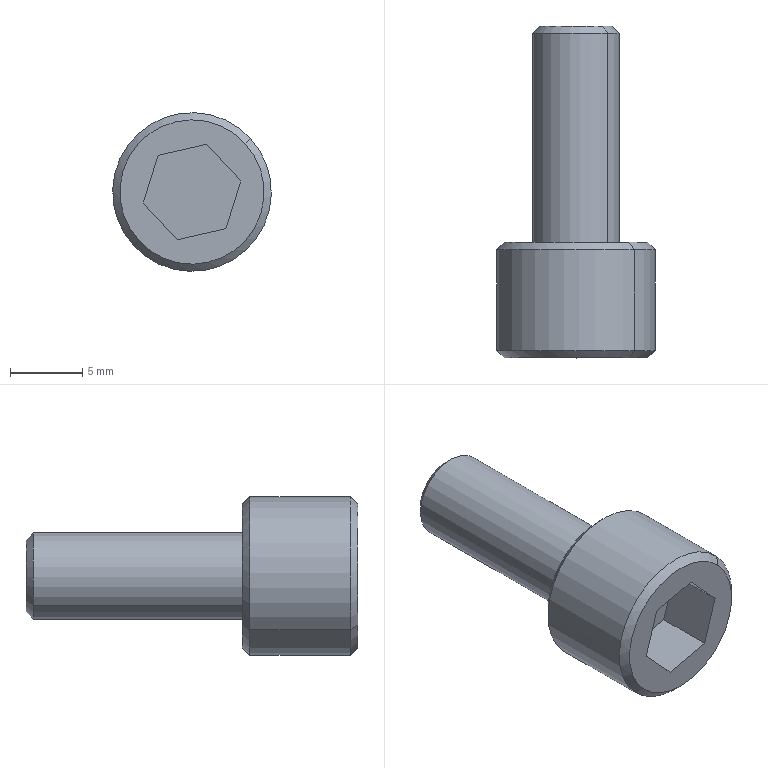Component | SolidWorks | 21-2 | 1 solid | 20 faces | box 11 x 23 x 11 mm | volume 1049 mm3 | plane 10 | cone 6 | cylinder 4 | commonest cylinder face diameters 6 x2 11 x2
STEP:
#1=CARTESIAN_POINT('',(-1.266,-2.358,0.6222));
#2=VERTEX_POINT('',#1);
#3=CARTESIAN_POINT('',(-1.121,-2.358,0.7558));
#4=VERTEX_POINT('',#3);
#5=CARTESIAN_POINT('',(-1.193,-2.358,0.689));
#6=DIRECTION('',(0.,1.,-0.));
#7=DIRECTION('',(-0.7345,0.,-0.6786));
#8=AXIS2_PLACEMENT_3D('',#5,#6,#7);
#9=CIRCLE('',#8,0.09843);
#10=EDGE_CURVE('',#2,#4,#9,.T.);
#11=ORIENTED_EDGE('',*,*,#10,.F.);
#12=CARTESIAN_POINT('',(-1.28,-2.377,0.6088));
#13=VERTEX_POINT('',#12);
#14=CARTESIAN_POINT('',(-1.266,-2.358,0.6222));
#15=DIRECTION('',(-0.5194,-0.7071,-0.4798));
#16=VECTOR('',#15,39.37);
#17=LINE('',#14,#16);
#18=EDGE_CURVE('',#2,#13,#17,.T.);
#19=ORIENTED_EDGE('',*,*,#18,.T.);
#20=CARTESIAN_POINT('',(-1.107,-2.377,0.7691));
#21=VERTEX_POINT('',#20);
#22=CARTESIAN_POINT('',(-1.193,-2.377,0.689));
#23=DIRECTION('',(-0.,-1.,0.));
#24=DIRECTION('',(-0.7345,0.,-0.6786));
#25=AXIS2_PLACEMENT_3D('',#22,#23,#24);
#26=CIRCLE('',#25,0.1181);
#27=EDGE_CURVE('',#21,#13,#26,.T.);
#28=ORIENTED_EDGE('',*,*,#27,.F.);
#29=CARTESIAN_POINT('',(-1.121,-2.358,0.7558));
#30=DIRECTION('',(0.5194,-0.7071,0.4798));
#31=VECTOR('',#30,39.37);
#32=LINE('',#29,#31);
#33=EDGE_CURVE('',#4,#21,#32,.T.);
#34=ORIENTED_EDGE('',*,*,#33,.F.);
#35=EDGE_LOOP('',(#11,#19,#28,#34));
#36=FACE_OUTER_BOUND('',#35,.T.);
#37=CARTESIAN_POINT('',(-1.193,-2.358,0.689));
#38=DIRECTION('',(-0.,-1.,0.));
#39=DIRECTION('',(0.7345,0.,0.6786));
#40=AXIS2_PLACEMENT_3D('',#37,#38,#39);
#41=CONICAL_SURFACE('',#40,0.09843,0.7854);
#42=ADVANCED_FACE('',(#36),#41,.T.);
#43=CARTESIAN_POINT('',(-1.338,-2.948,0.5554));
#44=VERTEX_POINT('',#43);
#45=CARTESIAN_POINT('',(-1.049,-2.948,0.8226));
#46=VERTEX_POINT('',#45);
#47=CARTESIAN_POINT('',(-1.193,-2.948,0.689));
#48=DIRECTION('',(0.,1.,-0.));
#49=DIRECTION('',(-0.7345,0.,-0.6786));
#50=AXIS2_PLACEMENT_3D('',#47,#48,#49);
#51=CIRCLE('',#50,0.1969);
#52=EDGE_CURVE('',#44,#46,#51,.T.);
#53=ORIENTED_EDGE('',*,*,#52,.F.);
#54=CARTESIAN_POINT('',(-1.352,-2.968,0.542));
#55=VERTEX_POINT('',#54);
#56=CARTESIAN_POINT('',(-1.338,-2.948,0.5554));
#57=DIRECTION('',(-0.5194,-0.7071,-0.4798));
#58=VECTOR('',#57,39.37);
#59=LINE('',#56,#58);
#60=EDGE_CURVE('',#44,#55,#59,.T.);
#61=ORIENTED_EDGE('',*,*,#60,.T.);
#62=CARTESIAN_POINT('',(-1.034,-2.968,0.8359));
#63=VERTEX_POINT('',#62);
#64=CARTESIAN_POINT('',(-1.193,-2.968,0.689));
#65=DIRECTION('',(-0.,-1.,0.));
#66=DIRECTION('',(-0.7345,0.,-0.6786));
#67=AXIS2_PLACEMENT_3D('',#64,#65,#66);
#68=CIRCLE('',#67,0.2165);
#69=EDGE_CURVE('',#63,#55,#68,.T.);
#70=ORIENTED_EDGE('',*,*,#69,.F.);
#71=CARTESIAN_POINT('',(-1.049,-2.948,0.8226));
#72=DIRECTION('',(0.5194,-0.7071,0.4798));
#73=VECTOR('',#72,39.37);
#74=LINE('',#71,#73);
#75=EDGE_CURVE('',#46,#63,#74,.T.);
#76=ORIENTED_EDGE('',*,*,#75,.F.);
#77=EDGE_LOOP('',(#53,#61,#70,#76));
#78=FACE_OUTER_BOUND('',#77,.T.);
#79=CARTESIAN_POINT('',(-1.193,-2.948,0.689));
#80=DIRECTION('',(-0.,-1.,0.));
#81=DIRECTION('',(0.7345,0.,0.6786));
#82=AXIS2_PLACEMENT_3D('',#79,#80,#81);
#83=CONICAL_SURFACE('',#82,0.1969,0.7854);
#84=ADVANCED_FACE('',(#78),#83,.T.);
#85=CARTESIAN_POINT('',(-1.049,-3.263,0.8226));
#86=VERTEX_POINT('',#85);
#87=CARTESIAN_POINT('',(-1.338,-3.263,0.5554));
#88=VERTEX_POINT('',#87);
#89=CARTESIAN_POINT('',(-1.193,-3.263,0.689));
#90=DIRECTION('',(-0.,-1.,0.));
#91=DIRECTION('',(-0.7345,0.,-0.6786));
#92=AXIS2_PLACEMENT_3D('',#89,#90,#91);
#93=CIRCLE('',#92,0.1969);
#94=EDGE_CURVE('',#86,#88,#93,.T.);
#95=ORIENTED_EDGE('',*,*,#94,.F.);
#96=CARTESIAN_POINT('',(-1.034,-3.243,0.8359));
#97=VERTEX_POINT('',#96);
#98=CARTESIAN_POINT('',(-1.034,-3.243,0.8359));
#99=DIRECTION('',(0.5194,0.7071,0.4798));
#100=VECTOR('',#99,39.37);
#101=LINE('',#98,#100);
#102=EDGE_CURVE('',#86,#97,#101,.T.);
#103=ORIENTED_EDGE('',*,*,#102,.T.);
#104=CARTESIAN_POINT('',(-1.352,-3.243,0.542));
#105=VERTEX_POINT('',#104);
#106=CARTESIAN_POINT('',(-1.193,-3.243,0.689));
#107=DIRECTION('',(0.,1.,-0.));
#108=DIRECTION('',(-0.7345,0.,-0.6786));
#109=AXIS2_PLACEMENT_3D('',#106,#107,#108);
#110=CIRCLE('',#109,0.2165);
#111=EDGE_CURVE('',#105,#97,#110,.T.);
#112=ORIENTED_EDGE('',*,*,#111,.F.);
#113=CARTESIAN_POINT('',(-1.352,-3.243,0.542));
#114=DIRECTION('',(-0.5194,0.7071,-0.4798));
#115=VECTOR('',#114,39.37);
#116=LINE('',#113,#115);
#117=EDGE_CURVE('',#88,#105,#116,.T.);
#118=ORIENTED_EDGE('',*,*,#117,.F.);
#119=EDGE_LOOP('',(#95,#103,#112,#118));
#120=FACE_OUTER_BOUND('',#119,.T.);
#121=CARTESIAN_POINT('',(-1.193,-3.243,0.689));
#122=DIRECTION('',(0.,1.,-0.));
#123=DIRECTION('',(-0.7345,0.,-0.6786));
#124=AXIS2_PLACEMENT_3D('',#121,#122,#123);
#125=CONICAL_SURFACE('',#124,0.2165,0.7854);
#126=ADVANCED_FACE('',(#120),#125,.T.);
#127=ORIENTED_EDGE('',*,*,#27,.T.);
#128=CARTESIAN_POINT('',(-1.28,-2.948,0.6088));
#129=VERTEX_POINT('',#128);
#130=CARTESIAN_POINT('',(-1.28,-2.358,0.6088));
#131=DIRECTION('',(-0.,-1.,0.));
#132=VECTOR('',#131,39.37);
#133=LINE('',#130,#132);
#134=EDGE_CURVE('',#13,#129,#133,.T.);
#135=ORIENTED_EDGE('',*,*,#134,.T.);
#136=CARTESIAN_POINT('',(-1.107,-2.948,0.7691));
#137=VERTEX_POINT('',#136);
#138=CARTESIAN_POINT('',(-1.193,-2.948,0.689));
#139=DIRECTION('',(0.,1.,-0.));
#140=DIRECTION('',(-0.7345,0.,-0.6786));
#141=AXIS2_PLACEMENT_3D('',#138,#139,#140);
#142=CIRCLE('',#141,0.1181);
#143=EDGE_CURVE('',#129,#137,#142,.T.);
#144=ORIENTED_EDGE('',*,*,#143,.T.);
#145=CARTESIAN_POINT('',(-1.107,-2.358,0.7691));
#146=DIRECTION('',(-0.,-1.,0.));
#147=VECTOR('',#146,39.37);
#148=LINE('',#145,#147);
#149=EDGE_CURVE('',#21,#137,#148,.T.);
#150=ORIENTED_EDGE('',*,*,#149,.F.);
#151=EDGE_LOOP('',(#127,#135,#144,#150));
#152=FACE_OUTER_BOUND('',#151,.T.);
#153=CARTESIAN_POINT('',(-1.193,-2.358,0.689));
#154=DIRECTION('',(-0.,-1.,0.));
#155=DIRECTION('',(0.7345,0.,0.6786));
#156=AXIS2_PLACEMENT_3D('',#153,#154,#155);
#157=CYLINDRICAL_SURFACE('',#156,0.1181);
#158=ADVANCED_FACE('',(#152),#157,.T.);
#159=ORIENTED_EDGE('',*,*,#69,.T.);
#160=CARTESIAN_POINT('',(-1.352,-2.948,0.542));
#161=DIRECTION('',(-0.,-1.,0.));
#162=VECTOR('',#161,39.37);
#163=LINE('',#160,#162);
#164=EDGE_CURVE('',#55,#105,#163,.T.);
#165=ORIENTED_EDGE('',*,*,#164,.T.);
#166=ORIENTED_EDGE('',*,*,#111,.T.);
#167=CARTESIAN_POINT('',(-1.034,-2.948,0.8359));
#168=DIRECTION('',(-0.,-1.,0.));
#169=VECTOR('',#168,39.37);
#170=LINE('',#167,#169);
#171=EDGE_CURVE('',#63,#97,#170,.T.);
#172=ORIENTED_EDGE('',*,*,#171,.F.);
#173=EDGE_LOOP('',(#159,#165,#166,#172));
#174=FACE_OUTER_BOUND('',#173,.T.);
#175=CARTESIAN_POINT('',(-1.193,-2.948,0.689));
#176=DIRECTION('',(-0.,-1.,0.));
#177=DIRECTION('',(0.7345,0.,0.6786));
#178=AXIS2_PLACEMENT_3D('',#175,#176,#177);
#179=CYLINDRICAL_SURFACE('',#178,0.2165);
#180=ADVANCED_FACE('',(#174),#179,.T.);
#181=ORIENTED_EDGE('',*,*,#164,.F.);
#182=CARTESIAN_POINT('',(-1.193,-2.968,0.689));
#183=DIRECTION('',(-0.,-1.,0.));
#184=DIRECTION('',(-0.7345,0.,-0.6786));
#185=AXIS2_PLACEMENT_3D('',#182,#183,#184);
#186=CIRCLE('',#185,0.2165);
#187=EDGE_CURVE('',#55,#63,#186,.T.);
#188=ORIENTED_EDGE('',*,*,#187,.T.);
#189=ORIENTED_EDGE('',*,*,#171,.T.);
#190=CARTESIAN_POINT('',(-1.193,-3.243,0.689));
#191=DIRECTION('',(0.,1.,-0.));
#192=DIRECTION('',(-0.7345,0.,-0.6786));
#193=AXIS2_PLACEMENT_3D('',#190,#191,#192);
#194=CIRCLE('',#193,0.2165);
#195=EDGE_CURVE('',#97,#105,#194,.T.);
#196=ORIENTED_EDGE('',*,*,#195,.T.);
#197=EDGE_LOOP('',(#181,#188,#189,#196));
#198=FACE_OUTER_BOUND('',#197,.T.);
#199=CARTESIAN_POINT('',(-1.193,-2.948,0.689));
#200=DIRECTION('',(-0.,-1.,0.));
#201=DIRECTION('',(0.7345,0.,0.6786));
#202=AXIS2_PLACEMENT_3D('',#199,#200,#201);
#203=CYLINDRICAL_SURFACE('',#202,0.2165);
#204=ADVANCED_FACE('',(#198),#203,.T.);
#205=CARTESIAN_POINT('',(-1.193,-2.948,0.689));
#206=DIRECTION('',(0.,1.,-0.));
#207=DIRECTION('',(-0.7345,0.,-0.6786));
#208=AXIS2_PLACEMENT_3D('',#205,#206,#207);
#209=CIRCLE('',#208,0.1969);
#210=EDGE_CURVE('',#46,#44,#209,.T.);
#211=ORIENTED_EDGE('',*,*,#210,.T.);
#212=ORIENTED_EDGE('',*,*,#52,.T.);
#213=EDGE_LOOP('',(#211,#212));
#214=FACE_OUTER_BOUND('',#213,.T.);
#215=CARTESIAN_POINT('',(-1.193,-2.948,0.689));
#216=DIRECTION('',(0.,1.,-0.));
#217=DIRECTION('',(-0.7345,0.,-0.6786));
#218=AXIS2_PLACEMENT_3D('',#215,#216,#217);
#219=CIRCLE('',#218,0.1181);
#220=EDGE_CURVE('',#137,#129,#219,.T.);
#221=ORIENTED_EDGE('',*,*,#220,.F.);
#222=ORIENTED_EDGE('',*,*,#143,.F.);
#223=EDGE_LOOP('',(#221,#222));
#224=FACE_BOUND('',#223,.T.);
#225=CARTESIAN_POINT('',(-1.193,-2.948,0.689));
#226=DIRECTION('',(0.,1.,-0.));
#227=DIRECTION('',(-0.7345,-0.,-0.6786));
#228=AXIS2_PLACEMENT_3D('',#225,#226,#227);
#229=PLANE('',#228);
#230=ADVANCED_FACE('',(#214,#224),#229,.T.);
#231=CARTESIAN_POINT('',(-1.06,-3.263,0.719));
#232=VERTEX_POINT('',#231);
#233=CARTESIAN_POINT('',(-1.153,-3.263,0.8192));
#234=VERTEX_POINT('',#233);
#235=CARTESIAN_POINT('',(-1.06,-3.263,0.719));
#236=DIRECTION('',(-0.6786,0.,0.7345));
#237=VECTOR('',#236,39.37);
#238=LINE('',#235,#237);
#239=EDGE_CURVE('',#232,#234,#238,.T.);
#240=ORIENTED_EDGE('',*,*,#239,.F.);
#241=CARTESIAN_POINT('',(-1.101,-3.263,0.5888));
#242=VERTEX_POINT('',#241);
#243=CARTESIAN_POINT('',(-1.101,-3.263,0.5888));
#244=DIRECTION('',(0.2968,0.,0.9549));
#245=VECTOR('',#244,39.37);
#246=LINE('',#243,#245);
#247=EDGE_CURVE('',#242,#232,#246,.T.);
#248=ORIENTED_EDGE('',*,*,#247,.F.);
#249=CARTESIAN_POINT('',(-1.234,-3.263,0.5587));
#250=VERTEX_POINT('',#249);
#251=CARTESIAN_POINT('',(-1.234,-3.263,0.5587));
#252=DIRECTION('',(0.9754,0.,0.2204));
#253=VECTOR('',#252,39.37);
#254=LINE('',#251,#253);
#255=EDGE_CURVE('',#250,#242,#254,.T.);
#256=ORIENTED_EDGE('',*,*,#255,.F.);
#257=CARTESIAN_POINT('',(-1.326,-3.263,0.6589));
#258=VERTEX_POINT('',#257);
#259=CARTESIAN_POINT('',(-1.326,-3.263,0.6589));
#260=DIRECTION('',(0.6786,-0.,-0.7345));
#261=VECTOR('',#260,39.37);
#262=LINE('',#259,#261);
#263=EDGE_CURVE('',#258,#250,#262,.T.);
#264=ORIENTED_EDGE('',*,*,#263,.F.);
#265=CARTESIAN_POINT('',(-1.286,-3.263,0.7892));
#266=VERTEX_POINT('',#265);
#267=CARTESIAN_POINT('',(-1.286,-3.263,0.7892));
#268=DIRECTION('',(-0.2968,-0.,-0.9549));
#269=VECTOR('',#268,39.37);
#270=LINE('',#267,#269);
#271=EDGE_CURVE('',#266,#258,#270,.T.);
#272=ORIENTED_EDGE('',*,*,#271,.F.);
#273=CARTESIAN_POINT('',(-1.153,-3.263,0.8192));
#274=DIRECTION('',(-0.9754,-0.,-0.2204));
#275=VECTOR('',#274,39.37);
#276=LINE('',#273,#275);
#277=EDGE_CURVE('',#234,#266,#276,.T.);
#278=ORIENTED_EDGE('',*,*,#277,.F.);
#279=EDGE_LOOP('',(#240,#248,#256,#264,#272,#278));
#280=FACE_BOUND('',#279,.T.);
#281=CARTESIAN_POINT('',(-1.193,-3.263,0.689));
#282=DIRECTION('',(-0.,-1.,0.));
#283=DIRECTION('',(-0.7345,0.,-0.6786));
#284=AXIS2_PLACEMENT_3D('',#281,#282,#283);
#285=CIRCLE('',#284,0.1969);
#286=EDGE_CURVE('',#88,#86,#285,.T.);
#287=ORIENTED_EDGE('',*,*,#286,.T.);
#288=ORIENTED_EDGE('',*,*,#94,.T.);
#289=EDGE_LOOP('',(#287,#288));
#290=FACE_OUTER_BOUND('',#289,.T.);
#291=CARTESIAN_POINT('',(-1.193,-3.263,0.689));
#292=DIRECTION('',(0.,1.,-0.));
#293=DIRECTION('',(-0.7345,-0.,-0.6786));
#294=AXIS2_PLACEMENT_3D('',#291,#292,#293);
#295=PLANE('',#294);
#296=ADVANCED_FACE('',(#280,#290),#295,.F.);
#297=ORIENTED_EDGE('',*,*,#134,.F.);
#298=CARTESIAN_POINT('',(-1.193,-2.377,0.689));
#299=DIRECTION('',(-0.,-1.,0.));
#300=DIRECTION('',(-0.7345,0.,-0.6786));
#301=AXIS2_PLACEMENT_3D('',#298,#299,#300);
#302=CIRCLE('',#301,0.1181);
#303=EDGE_CURVE('',#13,#21,#302,.T.);
#304=ORIENTED_EDGE('',*,*,#303,.T.);
#305=ORIENTED_EDGE('',*,*,#149,.T.);
#306=ORIENTED_EDGE('',*,*,#220,.T.);
#307=EDGE_LOOP('',(#297,#304,#305,#306));
#308=FACE_OUTER_BOUND('',#307,.T.);
#309=CARTESIAN_POINT('',(-1.193,-2.358,0.689));
#310=DIRECTION('',(-0.,-1.,0.));
#311=DIRECTION('',(0.7345,0.,0.6786));
#312=AXIS2_PLACEMENT_3D('',#309,#310,#311);
#313=CYLINDRICAL_SURFACE('',#312,0.1181);
#314=ADVANCED_FACE('',(#308),#313,.T.);
#315=CARTESIAN_POINT('',(-1.193,-2.358,0.689));
#316=DIRECTION('',(0.,1.,-0.));
#317=DIRECTION('',(-0.7345,0.,-0.6786));
#318=AXIS2_PLACEMENT_3D('',#315,#316,#317);
#319=CIRCLE('',#318,0.09843);
#320=EDGE_CURVE('',#4,#2,#319,.T.);
#321=ORIENTED_EDGE('',*,*,#320,.T.);
#322=ORIENTED_EDGE('',*,*,#10,.T.);
#323=EDGE_LOOP('',(#321,#322));
#324=FACE_OUTER_BOUND('',#323,.T.);
#325=CARTESIAN_POINT('',(-1.193,-2.358,0.689));
#326=DIRECTION('',(0.,1.,-0.));
#327=DIRECTION('',(-0.7345,-0.,-0.6786));
#328=AXIS2_PLACEMENT_3D('',#325,#326,#327);
#329=PLANE('',#328);
#330=ADVANCED_FACE('',(#324),#329,.T.);
#331=ORIENTED_EDGE('',*,*,#102,.F.);
#332=ORIENTED_EDGE('',*,*,#286,.F.);
#333=ORIENTED_EDGE('',*,*,#117,.T.);
#334=ORIENTED_EDGE('',*,*,#195,.F.);
#335=EDGE_LOOP('',(#331,#332,#333,#334));
#336=FACE_OUTER_BOUND('',#335,.T.);
#337=CARTESIAN_POINT('',(-1.193,-3.243,0.689));
#338=DIRECTION('',(0.,1.,-0.));
#339=DIRECTION('',(-0.7345,0.,-0.6786));
#340=AXIS2_PLACEMENT_3D('',#337,#338,#339);
#341=CONICAL_SURFACE('',#340,0.2165,0.7854);
#342=ADVANCED_FACE('',(#336),#341,.T.);
#343=ORIENTED_EDGE('',*,*,#60,.F.);
#344=ORIENTED_EDGE('',*,*,#210,.F.);
#345=ORIENTED_EDGE('',*,*,#75,.T.);
#346=ORIENTED_EDGE('',*,*,#187,.F.);
#347=EDGE_LOOP('',(#343,#344,#345,#346));
#348=FACE_OUTER_BOUND('',#347,.T.);
#349=CARTESIAN_POINT('',(-1.193,-2.948,0.689));
#350=DIRECTION('',(-0.,-1.,0.));
#351=DIRECTION('',(0.7345,0.,0.6786));
#352=AXIS2_PLACEMENT_3D('',#349,#350,#351);
#353=CONICAL_SURFACE('',#352,0.1969,0.7854);
#354=ADVANCED_FACE('',(#348),#353,.T.);
#355=ORIENTED_EDGE('',*,*,#18,.F.);
#356=ORIENTED_EDGE('',*,*,#320,.F.);
#357=ORIENTED_EDGE('',*,*,#33,.T.);
#358=ORIENTED_EDGE('',*,*,#303,.F.);
#359=EDGE_LOOP('',(#355,#356,#357,#358));
#360=FACE_OUTER_BOUND('',#359,.T.);
#361=CARTESIAN_POINT('',(-1.193,-2.358,0.689));
#362=DIRECTION('',(-0.,-1.,0.));
#363=DIRECTION('',(0.7345,0.,0.6786));
#364=AXIS2_PLACEMENT_3D('',#361,#362,#363);
#365=CONICAL_SURFACE('',#364,0.09843,0.7854);
#366=ADVANCED_FACE('',(#360),#365,.T.);
#367=ORIENTED_EDGE('',*,*,#247,.T.);
#368=CARTESIAN_POINT('',(-1.06,-3.106,0.719));
#369=VERTEX_POINT('',#368);
#370=CARTESIAN_POINT('',(-1.06,-3.106,0.719));
#371=DIRECTION('',(-0.,-1.,0.));
#372=VECTOR('',#371,39.37);
#373=LINE('',#370,#372);
#374=EDGE_CURVE('',#369,#232,#373,.T.);
#375=ORIENTED_EDGE('',*,*,#374,.F.);
#376=CARTESIAN_POINT('',(-1.101,-3.106,0.5888));
#377=VERTEX_POINT('',#376);
#378=CARTESIAN_POINT('',(-1.101,-3.106,0.5888));
#379=DIRECTION('',(0.2968,0.,0.9549));
#380=VECTOR('',#379,39.37);
#381=LINE('',#378,#380);
#382=EDGE_CURVE('',#377,#369,#381,.T.);
#383=ORIENTED_EDGE('',*,*,#382,.F.);
#384=CARTESIAN_POINT('',(-1.101,-3.106,0.5888));
#385=DIRECTION('',(-0.,-1.,0.));
#386=VECTOR('',#385,39.37);
#387=LINE('',#384,#386);
#388=EDGE_CURVE('',#377,#242,#387,.T.);
#389=ORIENTED_EDGE('',*,*,#388,.T.);
#390=EDGE_LOOP('',(#367,#375,#383,#389));
#391=FACE_OUTER_BOUND('',#390,.T.);
#392=CARTESIAN_POINT('',(-1.101,-3.106,0.5888));
#393=DIRECTION('',(0.9549,-0.,-0.2968));
#394=DIRECTION('',(-0.2968,-0.,-0.9549));
#395=AXIS2_PLACEMENT_3D('',#392,#393,#394);
#396=PLANE('',#395);
#397=ADVANCED_FACE('',(#391),#396,.F.);
#398=ORIENTED_EDGE('',*,*,#255,.T.);
#399=ORIENTED_EDGE('',*,*,#388,.F.);
#400=CARTESIAN_POINT('',(-1.234,-3.106,0.5587));
#401=VERTEX_POINT('',#400);
#402=CARTESIAN_POINT('',(-1.234,-3.106,0.5587));
#403=DIRECTION('',(0.9754,0.,0.2204));
#404=VECTOR('',#403,39.37);
#405=LINE('',#402,#404);
#406=EDGE_CURVE('',#401,#377,#405,.T.);
#407=ORIENTED_EDGE('',*,*,#406,.F.);
#408=CARTESIAN_POINT('',(-1.234,-3.106,0.5587));
#409=DIRECTION('',(-0.,-1.,0.));
#410=VECTOR('',#409,39.37);
#411=LINE('',#408,#410);
#412=EDGE_CURVE('',#401,#250,#411,.T.);
#413=ORIENTED_EDGE('',*,*,#412,.T.);
#414=EDGE_LOOP('',(#398,#399,#407,#413));
#415=FACE_OUTER_BOUND('',#414,.T.);
#416=CARTESIAN_POINT('',(-1.234,-3.106,0.5587));
#417=DIRECTION('',(0.2204,-0.,-0.9754));
#418=DIRECTION('',(-0.9754,-0.,-0.2204));
#419=AXIS2_PLACEMENT_3D('',#416,#417,#418);
#420=PLANE('',#419);
#421=ADVANCED_FACE('',(#415),#420,.F.);
#422=ORIENTED_EDGE('',*,*,#263,.T.);
#423=ORIENTED_EDGE('',*,*,#412,.F.);
#424=CARTESIAN_POINT('',(-1.326,-3.106,0.6589));
#425=VERTEX_POINT('',#424);
#426=CARTESIAN_POINT('',(-1.326,-3.106,0.6589));
#427=DIRECTION('',(0.6786,-0.,-0.7345));
#428=VECTOR('',#427,39.37);
#429=LINE('',#426,#428);
#430=EDGE_CURVE('',#425,#401,#429,.T.);
#431=ORIENTED_EDGE('',*,*,#430,.F.);
#432=CARTESIAN_POINT('',(-1.326,-3.106,0.6589));
#433=DIRECTION('',(-0.,-1.,0.));
#434=VECTOR('',#433,39.37);
#435=LINE('',#432,#434);
#436=EDGE_CURVE('',#425,#258,#435,.T.);
#437=ORIENTED_EDGE('',*,*,#436,.T.);
#438=EDGE_LOOP('',(#422,#423,#431,#437));
#439=FACE_OUTER_BOUND('',#438,.T.);
#440=CARTESIAN_POINT('',(-1.326,-3.106,0.6589));
#441=DIRECTION('',(-0.7345,-0.,-0.6786));
#442=DIRECTION('',(-0.6786,0.,0.7345));
#443=AXIS2_PLACEMENT_3D('',#440,#441,#442);
#444=PLANE('',#443);
#445=ADVANCED_FACE('',(#439),#444,.F.);
#446=ORIENTED_EDGE('',*,*,#271,.T.);
#447=ORIENTED_EDGE('',*,*,#436,.F.);
#448=CARTESIAN_POINT('',(-1.286,-3.106,0.7892));
#449=VERTEX_POINT('',#448);
#450=CARTESIAN_POINT('',(-1.286,-3.106,0.7892));
#451=DIRECTION('',(-0.2968,-0.,-0.9549));
#452=VECTOR('',#451,39.37);
#453=LINE('',#450,#452);
#454=EDGE_CURVE('',#449,#425,#453,.T.);
#455=ORIENTED_EDGE('',*,*,#454,.F.);
#456=CARTESIAN_POINT('',(-1.286,-3.106,0.7892));
#457=DIRECTION('',(-0.,-1.,0.));
#458=VECTOR('',#457,39.37);
#459=LINE('',#456,#458);
#460=EDGE_CURVE('',#449,#266,#459,.T.);
#461=ORIENTED_EDGE('',*,*,#460,.T.);
#462=EDGE_LOOP('',(#446,#447,#455,#461));
#463=FACE_OUTER_BOUND('',#462,.T.);
#464=CARTESIAN_POINT('',(-1.286,-3.106,0.7892));
#465=DIRECTION('',(-0.9549,0.,0.2968));
#466=DIRECTION('',(0.2968,0.,0.9549));
#467=AXIS2_PLACEMENT_3D('',#464,#465,#466);
#468=PLANE('',#467);
#469=ADVANCED_FACE('',(#463),#468,.F.);
#470=ORIENTED_EDGE('',*,*,#277,.T.);
#471=ORIENTED_EDGE('',*,*,#460,.F.);
#472=CARTESIAN_POINT('',(-1.153,-3.106,0.8192));
#473=VERTEX_POINT('',#472);
#474=CARTESIAN_POINT('',(-1.153,-3.106,0.8192));
#475=DIRECTION('',(-0.9754,-0.,-0.2204));
#476=VECTOR('',#475,39.37);
#477=LINE('',#474,#476);
#478=EDGE_CURVE('',#473,#449,#477,.T.);
#479=ORIENTED_EDGE('',*,*,#478,.F.);
#480=CARTESIAN_POINT('',(-1.153,-3.106,0.8192));
#481=DIRECTION('',(-0.,-1.,0.));
#482=VECTOR('',#481,39.37);
#483=LINE('',#480,#482);
#484=EDGE_CURVE('',#473,#234,#483,.T.);
#485=ORIENTED_EDGE('',*,*,#484,.T.);
#486=EDGE_LOOP('',(#470,#471,#479,#485));
#487=FACE_OUTER_BOUND('',#486,.T.);
#488=CARTESIAN_POINT('',(-1.153,-3.106,0.8192));
#489=DIRECTION('',(-0.2204,0.,0.9754));
#490=DIRECTION('',(0.9754,0.,0.2204));
#491=AXIS2_PLACEMENT_3D('',#488,#489,#490);
#492=PLANE('',#491);
#493=ADVANCED_FACE('',(#487),#492,.F.);
#494=ORIENTED_EDGE('',*,*,#239,.T.);
#495=ORIENTED_EDGE('',*,*,#484,.F.);
#496=CARTESIAN_POINT('',(-1.06,-3.106,0.719));
#497=DIRECTION('',(-0.6786,0.,0.7345));
#498=VECTOR('',#497,39.37);
#499=LINE('',#496,#498);
#500=EDGE_CURVE('',#369,#473,#499,.T.);
#501=ORIENTED_EDGE('',*,*,#500,.F.);
#502=ORIENTED_EDGE('',*,*,#374,.T.);
#503=EDGE_LOOP('',(#494,#495,#501,#502));
#504=FACE_OUTER_BOUND('',#503,.T.);
#505=CARTESIAN_POINT('',(-1.06,-3.106,0.719));
#506=DIRECTION('',(0.7345,0.,0.6786));
#507=DIRECTION('',(0.6786,-0.,-0.7345));
#508=AXIS2_PLACEMENT_3D('',#505,#506,#507);
#509=PLANE('',#508);
#510=ADVANCED_FACE('',(#504),#509,.F.);
#511=ORIENTED_EDGE('',*,*,#382,.T.);
#512=ORIENTED_EDGE('',*,*,#500,.T.);
#513=ORIENTED_EDGE('',*,*,#478,.T.);
#514=ORIENTED_EDGE('',*,*,#454,.T.);
#515=ORIENTED_EDGE('',*,*,#430,.T.);
#516=ORIENTED_EDGE('',*,*,#406,.T.);
#517=EDGE_LOOP('',(#511,#512,#513,#514,#515,#516));
#518=FACE_OUTER_BOUND('',#517,.T.);
#519=CARTESIAN_POINT('',(-1.193,-3.106,0.689));
#520=DIRECTION('',(-0.,-1.,0.));
#521=DIRECTION('',(0.7345,0.,0.6786));
#522=AXIS2_PLACEMENT_3D('',#519,#520,#521);
#523=PLANE('',#522);
#524=ADVANCED_FACE('',(#518),#523,.T.);
#525=CLOSED_SHELL('',(#42,#84,#126,#158,#180,#204,#230,#296,#314,#330,#342,#354,#366,#397,#421,#445,#469,#493,#510,#524));
#526=MANIFOLD_SOLID_BREP('',#525);
#527=CARTESIAN_POINT('',(0.,0.,0.));
#528=DIRECTION('',(0.,0.,1.));
#529=DIRECTION('',(1.,0.,0.));
#530=AXIS2_PLACEMENT_3D('',#527,#528,#529);
#531=(LENGTH_UNIT()NAMED_UNIT(*)SI_UNIT($,.METRE.));
#532=LENGTH_MEASURE_WITH_UNIT(LENGTH_MEASURE(0.0254),#531);
#533=DIMENSIONAL_EXPONENTS(1.,0.,0.,0.,0.,0.,0.);
#534=(CONVERSION_BASED_UNIT('',#532)LENGTH_UNIT()NAMED_UNIT(#533));
#535=UNCERTAINTY_MEASURE_WITH_UNIT(LENGTH_MEASURE(0.00001),#534,'','');
#536=(NAMED_UNIT(*)PLANE_ANGLE_UNIT()SI_UNIT($,.RADIAN.));
#537=(NAMED_UNIT(*)SI_UNIT($,.STERADIAN.)SOLID_ANGLE_UNIT());
#538=(GEOMETRIC_REPRESENTATION_CONTEXT(3)GLOBAL_UNCERTAINTY_ASSIGNED_CONTEXT((#535))GLOBAL_UNIT_ASSIGNED_CONTEXT((#534,#536,#537))REPRESENTATION_CONTEXT('',''));
#539=ADVANCED_BREP_SHAPE_REPRESENTATION('',(#526,#530),#538);
#540=COLOUR_RGB('',0.7922,0.8196,0.9333);
#541=FILL_AREA_STYLE_COLOUR('',#540);
#542=FILL_AREA_STYLE('',(#541));
#543=SURFACE_STYLE_FILL_AREA(#542);
#544=SURFACE_SIDE_STYLE('',(#543));
#545=SURFACE_STYLE_USAGE(.BOTH.,#544);
#546=PRESENTATION_STYLE_ASSIGNMENT((#545));
#547=STYLED_ITEM('',(#546),#526);
#548=PRESENTATION_LAYER_ASSIGNMENT('','',(#547));
#549=(LENGTH_UNIT()NAMED_UNIT(*)SI_UNIT($,.METRE.));
#550=LENGTH_MEASURE_WITH_UNIT(LENGTH_MEASURE(0.0254),#549);
#551=DIMENSIONAL_EXPONENTS(1.,0.,0.,0.,0.,0.,0.);
#552=(CONVERSION_BASED_UNIT('',#550)LENGTH_UNIT()NAMED_UNIT(#551));
#553=UNCERTAINTY_MEASURE_WITH_UNIT(LENGTH_MEASURE(0.00001),#552,'','');
#554=(NAMED_UNIT(*)PLANE_ANGLE_UNIT()SI_UNIT($,.RADIAN.));
#555=(NAMED_UNIT(*)SI_UNIT($,.STERADIAN.)SOLID_ANGLE_UNIT());
#556=(GEOMETRIC_REPRESENTATION_CONTEXT(3)GLOBAL_UNCERTAINTY_ASSIGNED_CONTEXT((#553))GLOBAL_UNIT_ASSIGNED_CONTEXT((#552,#554,#555))REPRESENTATION_CONTEXT('',''));
#557=MECHANICAL_DESIGN_GEOMETRIC_PRESENTATION_REPRESENTATION('',(#547),#556);